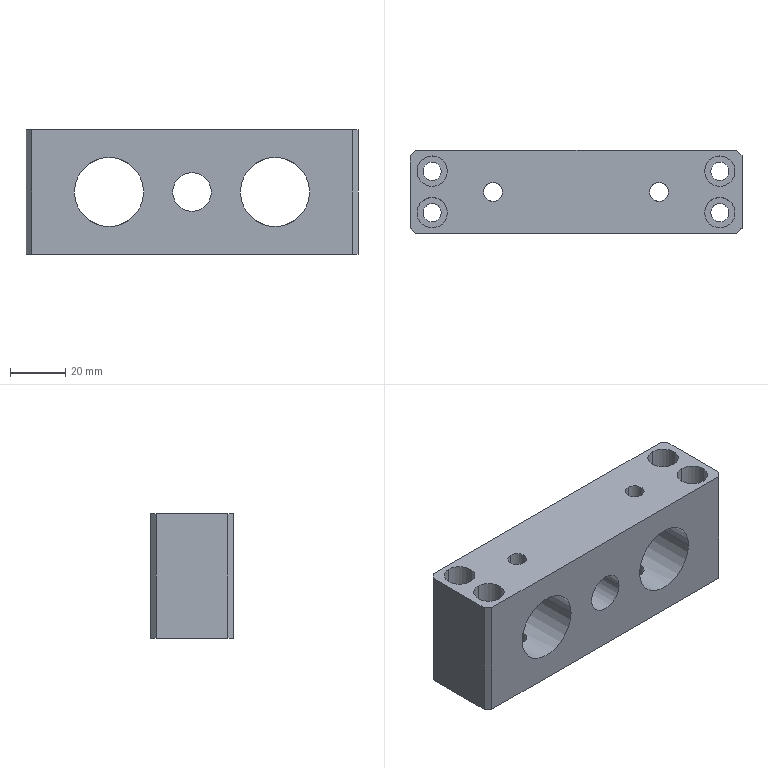Component | SolidWorks | CCDJSHeightAdjustmentBlock01-1 | 1 solid | 44 faces | box 120 x 30 x 45 mm | volume 112643 mm3 | cylinder 30 | plane 14 | commonest cylinder face diameters 11 x8 6.6 x8 6.8 x8 25 x4 14 x2 | material A6061
build123d program:
from build123d import *

# Parameters (mm, degrees)
SKETCH1_W                                       = 120
SKETCH1_H                                       = 45
BOSS_EXTRUDE1_DEPTH                             = 30
SKETCH2_R                                       = 12.5
CUT_EXTRUDE1_DEPTH                              = 35
SKETCH4_R                                       = 6
CUT_EXTRUDE3_DEPTH                              = 39
M8_TAPPED_HOLE1_D                               = 6.8
M6_HEX_SOCKET_HEAD_CAP_SCREW_CBORE1_D           = 6.6
M6_HEX_SOCKET_HEAD_CAP_SCREW_CBORE1_CBORE_D     = 11
M6_HEX_SOCKET_HEAD_CAP_SCREW_CBORE1_CBORE_DEPTH = 30
CHAMFER1_SIZE                                   = 2
M16_TAPPED_HOLE1_D                              = 14
M16_TAPPED_HOLE1_DEPTH                          = 38
M16_TAPPED_HOLE1_TIP                            = 4.206


with BuildPart() as part:
    # Sketch1 → Boss-Extrude1 (new body)
    with BuildSketch(Plane.XY):
        Rectangle(SKETCH1_W, SKETCH1_H)
    extrude(amount=BOSS_EXTRUDE1_DEPTH)

    # Sketch2 → Cut-Extrude1 (cut)
    with BuildSketch(Plane.XY.offset(30)):
        with Locations((-30, 0)):
            Circle(SKETCH2_R)
        with Locations(Location((30, 0, 0), (0, 0, 180))):
            Circle(SKETCH2_R)
    extrude(amount=-CUT_EXTRUDE1_DEPTH, mode=Mode.SUBTRACT)

    # Sketch4 → Cut-Extrude3 (cut)
    with BuildSketch(Plane.XY.offset(30)):
        Circle(SKETCH4_R)
    extrude(amount=-CUT_EXTRUDE3_DEPTH, mode=Mode.SUBTRACT)

    # M8 Tapped Hole1 (through all)
    with Locations(Plane(origin=(0, -22.5, 0), x_dir=(-1, 0, 0), z_dir=(0, -1, 0))):
        with Locations((-30, -15), (30, -15)):
            Hole(M8_TAPPED_HOLE1_D / 2)

    # M6 Hex Socket Head Cap Screw CBORE1 (through all)
    with Locations(Plane(origin=(0, -22.5, 0), x_dir=(-1, 0, 0), z_dir=(0, -1, 0))):
        with Locations((-52, -22.5), (52, -22.5), (52, -7.5), (-52, -7.5)):
            CounterBoreHole(M6_HEX_SOCKET_HEAD_CAP_SCREW_CBORE1_D / 2, M6_HEX_SOCKET_HEAD_CAP_SCREW_CBORE1_CBORE_D / 2, M6_HEX_SOCKET_HEAD_CAP_SCREW_CBORE1_CBORE_DEPTH)

    # Chamfer1
    chamfer1_edges = [part.edges().sort_by_distance(p)[0] for p in [
        (-60, 0, 30),
        (60, 0, 30),
        (-60, 0, 0),
        (60, 0, 0),
    ]]
    chamfer(chamfer1_edges, length=CHAMFER1_SIZE)

    # M16 Tapped Hole1
    with Locations(Plane.XY.offset(30)):
        with Locations((0, 0)):
            Hole(M16_TAPPED_HOLE1_D / 2, depth=M16_TAPPED_HOLE1_DEPTH)
            with Locations((0, 0, -(M16_TAPPED_HOLE1_DEPTH + M16_TAPPED_HOLE1_TIP / 2))):  # 118° drill point
                Cone(0, M16_TAPPED_HOLE1_D / 2, M16_TAPPED_HOLE1_TIP, mode=Mode.SUBTRACT)


solid = part.part

# Placed as in the assembly
solid = solid.moved(Location((0, 411.564, 0), (-90, 0, 0)))